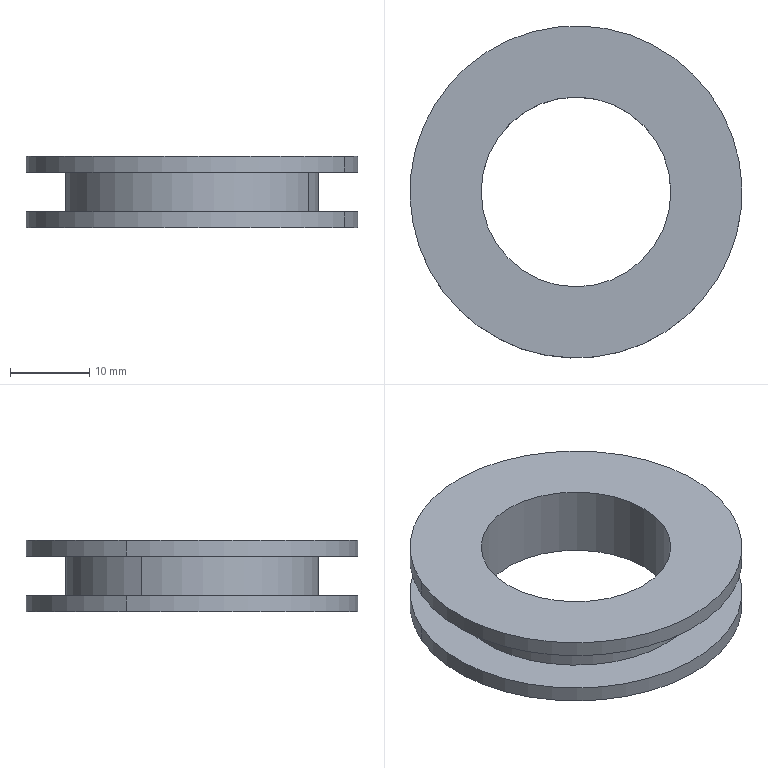Component | SolidWorks | PulleyAssembly-1_Pulley-1 | 1 solid | 12 faces | box 42 x 42 x 9 mm | volume 5492 mm3 | cylinder 8 | plane 4 | commonest cylinder face diameters 42 x4 32 x2 24 x2
build123d program:
from build123d import *


with BuildPart() as part:
    # Sketch1 → Revolve1 (revolve)
    with BuildSketch(Plane(origin=(0, 0, 0), x_dir=(1, 0, 0), z_dir=(0, 1, 0)), mode=Mode.PRIVATE) as revolve1_sk:
        Polygon((12, 4.5), (21, 4.5), (21, 2.5), (16, 2.5), (16, -2.5), (21, -2.5), (21, -4.5), (12, -4.5), align=None)
    revolve(revolve1_sk.sketch.rotate(Axis((0, 0, -4.95), (0, 0, 1)), 180), axis=Axis((0, 0, -4.95), (0, 0, 1)))


solid = part.part

# Placed as in the assembly
solid = solid.moved(Location((-354.55, -345.434, 489.481), (0, 0, 0)))
STEP:
#1=CARTESIAN_POINT('',(-14.718,-13.273,19.094));
#2=VERTEX_POINT('',#1);
#3=CARTESIAN_POINT('',(-13.199,-13.927,19.094));
#4=VERTEX_POINT('',#3);
#5=CARTESIAN_POINT('',(-13.959,-13.6,19.094));
#6=DIRECTION('',(-0.,0.,1.));
#7=DIRECTION('',(-0.9185,0.3954,0.));
#8=AXIS2_PLACEMENT_3D('',#5,#6,#7);
#9=CIRCLE('',#8,0.8268);
#10=EDGE_CURVE('',#2,#4,#9,.T.);
#11=ORIENTED_EDGE('',*,*,#10,.T.);
#12=CARTESIAN_POINT('',(-13.199,-13.927,19.172));
#13=VERTEX_POINT('',#12);
#14=CARTESIAN_POINT('',(-13.199,-13.927,19.466));
#15=DIRECTION('',(-0.,0.,1.));
#16=VECTOR('',#15,39.37);
#17=LINE('',#14,#16);
#18=EDGE_CURVE('',#4,#13,#17,.T.);
#19=ORIENTED_EDGE('',*,*,#18,.T.);
#20=CARTESIAN_POINT('',(-14.718,-13.273,19.172));
#21=VERTEX_POINT('',#20);
#22=CARTESIAN_POINT('',(-13.959,-13.6,19.172));
#23=DIRECTION('',(-0.,0.,1.));
#24=DIRECTION('',(-0.9185,0.3954,0.));
#25=AXIS2_PLACEMENT_3D('',#22,#23,#24);
#26=CIRCLE('',#25,0.8268);
#27=EDGE_CURVE('',#21,#13,#26,.T.);
#28=ORIENTED_EDGE('',*,*,#27,.F.);
#29=CARTESIAN_POINT('',(-14.718,-13.273,19.466));
#30=DIRECTION('',(-0.,0.,1.));
#31=VECTOR('',#30,39.37);
#32=LINE('',#29,#31);
#33=EDGE_CURVE('',#2,#21,#32,.T.);
#34=ORIENTED_EDGE('',*,*,#33,.F.);
#35=EDGE_LOOP('',(#11,#19,#28,#34));
#36=FACE_OUTER_BOUND('',#35,.T.);
#37=CARTESIAN_POINT('',(-13.959,-13.6,19.466));
#38=DIRECTION('',(-0.,0.,1.));
#39=DIRECTION('',(-0.9185,0.3954,0.));
#40=AXIS2_PLACEMENT_3D('',#37,#38,#39);
#41=CYLINDRICAL_SURFACE('',#40,0.8268);
#42=ADVANCED_FACE('',(#36),#41,.T.);
#43=CARTESIAN_POINT('',(-14.537,-13.351,19.172));
#44=VERTEX_POINT('',#43);
#45=CARTESIAN_POINT('',(-13.38,-13.849,19.172));
#46=VERTEX_POINT('',#45);
#47=CARTESIAN_POINT('',(-13.959,-13.6,19.172));
#48=DIRECTION('',(-0.,0.,1.));
#49=DIRECTION('',(-0.9185,0.3954,0.));
#50=AXIS2_PLACEMENT_3D('',#47,#48,#49);
#51=CIRCLE('',#50,0.6299);
#52=EDGE_CURVE('',#44,#46,#51,.T.);
#53=ORIENTED_EDGE('',*,*,#52,.T.);
#54=CARTESIAN_POINT('',(-13.38,-13.849,19.369));
#55=VERTEX_POINT('',#54);
#56=CARTESIAN_POINT('',(-13.38,-13.849,19.466));
#57=DIRECTION('',(-0.,0.,1.));
#58=VECTOR('',#57,39.37);
#59=LINE('',#56,#58);
#60=EDGE_CURVE('',#46,#55,#59,.T.);
#61=ORIENTED_EDGE('',*,*,#60,.T.);
#62=CARTESIAN_POINT('',(-14.537,-13.351,19.369));
#63=VERTEX_POINT('',#62);
#64=CARTESIAN_POINT('',(-13.959,-13.6,19.369));
#65=DIRECTION('',(-0.,0.,1.));
#66=DIRECTION('',(-0.9185,0.3954,0.));
#67=AXIS2_PLACEMENT_3D('',#64,#65,#66);
#68=CIRCLE('',#67,0.6299);
#69=EDGE_CURVE('',#63,#55,#68,.T.);
#70=ORIENTED_EDGE('',*,*,#69,.F.);
#71=CARTESIAN_POINT('',(-14.537,-13.351,19.466));
#72=DIRECTION('',(-0.,0.,1.));
#73=VECTOR('',#72,39.37);
#74=LINE('',#71,#73);
#75=EDGE_CURVE('',#44,#63,#74,.T.);
#76=ORIENTED_EDGE('',*,*,#75,.F.);
#77=EDGE_LOOP('',(#53,#61,#70,#76));
#78=FACE_OUTER_BOUND('',#77,.T.);
#79=CARTESIAN_POINT('',(-13.959,-13.6,19.466));
#80=DIRECTION('',(-0.,0.,1.));
#81=DIRECTION('',(-0.9185,0.3954,0.));
#82=AXIS2_PLACEMENT_3D('',#79,#80,#81);
#83=CYLINDRICAL_SURFACE('',#82,0.6299);
#84=ADVANCED_FACE('',(#78),#83,.T.);
#85=CARTESIAN_POINT('',(-14.718,-13.273,19.369));
#86=VERTEX_POINT('',#85);
#87=CARTESIAN_POINT('',(-13.199,-13.927,19.369));
#88=VERTEX_POINT('',#87);
#89=CARTESIAN_POINT('',(-13.959,-13.6,19.369));
#90=DIRECTION('',(-0.,0.,1.));
#91=DIRECTION('',(-0.9185,0.3954,0.));
#92=AXIS2_PLACEMENT_3D('',#89,#90,#91);
#93=CIRCLE('',#92,0.8268);
#94=EDGE_CURVE('',#86,#88,#93,.T.);
#95=ORIENTED_EDGE('',*,*,#94,.T.);
#96=CARTESIAN_POINT('',(-13.199,-13.927,19.448));
#97=VERTEX_POINT('',#96);
#98=CARTESIAN_POINT('',(-13.199,-13.927,19.466));
#99=DIRECTION('',(-0.,0.,1.));
#100=VECTOR('',#99,39.37);
#101=LINE('',#98,#100);
#102=EDGE_CURVE('',#88,#97,#101,.T.);
#103=ORIENTED_EDGE('',*,*,#102,.T.);
#104=CARTESIAN_POINT('',(-14.718,-13.273,19.448));
#105=VERTEX_POINT('',#104);
#106=CARTESIAN_POINT('',(-13.959,-13.6,19.448));
#107=DIRECTION('',(-0.,0.,1.));
#108=DIRECTION('',(-0.9185,0.3954,0.));
#109=AXIS2_PLACEMENT_3D('',#106,#107,#108);
#110=CIRCLE('',#109,0.8268);
#111=EDGE_CURVE('',#105,#97,#110,.T.);
#112=ORIENTED_EDGE('',*,*,#111,.F.);
#113=CARTESIAN_POINT('',(-14.718,-13.273,19.466));
#114=DIRECTION('',(-0.,0.,1.));
#115=VECTOR('',#114,39.37);
#116=LINE('',#113,#115);
#117=EDGE_CURVE('',#86,#105,#116,.T.);
#118=ORIENTED_EDGE('',*,*,#117,.F.);
#119=EDGE_LOOP('',(#95,#103,#112,#118));
#120=FACE_OUTER_BOUND('',#119,.T.);
#121=CARTESIAN_POINT('',(-13.959,-13.6,19.466));
#122=DIRECTION('',(-0.,0.,1.));
#123=DIRECTION('',(-0.9185,0.3954,0.));
#124=AXIS2_PLACEMENT_3D('',#121,#122,#123);
#125=CYLINDRICAL_SURFACE('',#124,0.8268);
#126=ADVANCED_FACE('',(#120),#125,.T.);
#127=CARTESIAN_POINT('',(-13.525,-13.787,19.094));
#128=VERTEX_POINT('',#127);
#129=CARTESIAN_POINT('',(-14.393,-13.413,19.094));
#130=VERTEX_POINT('',#129);
#131=CARTESIAN_POINT('',(-13.959,-13.6,19.094));
#132=DIRECTION('',(-0.,0.,1.));
#133=DIRECTION('',(-0.9185,0.3954,0.));
#134=AXIS2_PLACEMENT_3D('',#131,#132,#133);
#135=CIRCLE('',#134,0.4724);
#136=EDGE_CURVE('',#128,#130,#135,.T.);
#137=ORIENTED_EDGE('',*,*,#136,.F.);
#138=CARTESIAN_POINT('',(-13.525,-13.787,19.448));
#139=VERTEX_POINT('',#138);
#140=CARTESIAN_POINT('',(-13.525,-13.787,19.466));
#141=DIRECTION('',(-0.,0.,1.));
#142=VECTOR('',#141,39.37);
#143=LINE('',#140,#142);
#144=EDGE_CURVE('',#128,#139,#143,.T.);
#145=ORIENTED_EDGE('',*,*,#144,.T.);
#146=CARTESIAN_POINT('',(-14.393,-13.413,19.448));
#147=VERTEX_POINT('',#146);
#148=CARTESIAN_POINT('',(-13.959,-13.6,19.448));
#149=DIRECTION('',(-0.,0.,1.));
#150=DIRECTION('',(-0.9185,0.3954,0.));
#151=AXIS2_PLACEMENT_3D('',#148,#149,#150);
#152=CIRCLE('',#151,0.4724);
#153=EDGE_CURVE('',#139,#147,#152,.T.);
#154=ORIENTED_EDGE('',*,*,#153,.T.);
#155=CARTESIAN_POINT('',(-14.393,-13.413,19.466));
#156=DIRECTION('',(-0.,0.,1.));
#157=VECTOR('',#156,39.37);
#158=LINE('',#155,#157);
#159=EDGE_CURVE('',#130,#147,#158,.T.);
#160=ORIENTED_EDGE('',*,*,#159,.F.);
#161=EDGE_LOOP('',(#137,#145,#154,#160));
#162=FACE_OUTER_BOUND('',#161,.T.);
#163=CARTESIAN_POINT('',(-13.959,-13.6,19.466));
#164=DIRECTION('',(-0.,0.,1.));
#165=DIRECTION('',(-0.9185,0.3954,0.));
#166=AXIS2_PLACEMENT_3D('',#163,#164,#165);
#167=CYLINDRICAL_SURFACE('',#166,0.4724);
#168=ADVANCED_FACE('',(#162),#167,.F.);
#169=ORIENTED_EDGE('',*,*,#144,.F.);
#170=CARTESIAN_POINT('',(-13.959,-13.6,19.094));
#171=DIRECTION('',(-0.,0.,1.));
#172=DIRECTION('',(-0.9185,0.3954,0.));
#173=AXIS2_PLACEMENT_3D('',#170,#171,#172);
#174=CIRCLE('',#173,0.4724);
#175=EDGE_CURVE('',#130,#128,#174,.T.);
#176=ORIENTED_EDGE('',*,*,#175,.F.);
#177=ORIENTED_EDGE('',*,*,#159,.T.);
#178=CARTESIAN_POINT('',(-13.959,-13.6,19.448));
#179=DIRECTION('',(-0.,0.,1.));
#180=DIRECTION('',(-0.9185,0.3954,0.));
#181=AXIS2_PLACEMENT_3D('',#178,#179,#180);
#182=CIRCLE('',#181,0.4724);
#183=EDGE_CURVE('',#147,#139,#182,.T.);
#184=ORIENTED_EDGE('',*,*,#183,.T.);
#185=EDGE_LOOP('',(#169,#176,#177,#184));
#186=FACE_OUTER_BOUND('',#185,.T.);
#187=CARTESIAN_POINT('',(-13.959,-13.6,19.466));
#188=DIRECTION('',(-0.,0.,1.));
#189=DIRECTION('',(-0.9185,0.3954,0.));
#190=AXIS2_PLACEMENT_3D('',#187,#188,#189);
#191=CYLINDRICAL_SURFACE('',#190,0.4724);
#192=ADVANCED_FACE('',(#186),#191,.F.);
#193=ORIENTED_EDGE('',*,*,#183,.F.);
#194=ORIENTED_EDGE('',*,*,#153,.F.);
#195=EDGE_LOOP('',(#193,#194));
#196=FACE_BOUND('',#195,.T.);
#197=ORIENTED_EDGE('',*,*,#111,.T.);
#198=CARTESIAN_POINT('',(-13.959,-13.6,19.448));
#199=DIRECTION('',(-0.,0.,1.));
#200=DIRECTION('',(-0.9185,0.3954,0.));
#201=AXIS2_PLACEMENT_3D('',#198,#199,#200);
#202=CIRCLE('',#201,0.8268);
#203=EDGE_CURVE('',#97,#105,#202,.T.);
#204=ORIENTED_EDGE('',*,*,#203,.T.);
#205=EDGE_LOOP('',(#197,#204));
#206=FACE_OUTER_BOUND('',#205,.T.);
#207=CARTESIAN_POINT('',(-13.525,-13.787,19.448));
#208=DIRECTION('',(0.,-0.,-1.));
#209=DIRECTION('',(0.9185,-0.3954,0.));
#210=AXIS2_PLACEMENT_3D('',#207,#208,#209);
#211=PLANE('',#210);
#212=ADVANCED_FACE('',(#196,#206),#211,.F.);
#213=ORIENTED_EDGE('',*,*,#102,.F.);
#214=CARTESIAN_POINT('',(-13.959,-13.6,19.369));
#215=DIRECTION('',(-0.,0.,1.));
#216=DIRECTION('',(-0.9185,0.3954,0.));
#217=AXIS2_PLACEMENT_3D('',#214,#215,#216);
#218=CIRCLE('',#217,0.8268);
#219=EDGE_CURVE('',#88,#86,#218,.T.);
#220=ORIENTED_EDGE('',*,*,#219,.T.);
#221=ORIENTED_EDGE('',*,*,#117,.T.);
#222=ORIENTED_EDGE('',*,*,#203,.F.);
#223=EDGE_LOOP('',(#213,#220,#221,#222));
#224=FACE_OUTER_BOUND('',#223,.T.);
#225=CARTESIAN_POINT('',(-13.959,-13.6,19.466));
#226=DIRECTION('',(-0.,0.,1.));
#227=DIRECTION('',(-0.9185,0.3954,0.));
#228=AXIS2_PLACEMENT_3D('',#225,#226,#227);
#229=CYLINDRICAL_SURFACE('',#228,0.8268);
#230=ADVANCED_FACE('',(#224),#229,.T.);
#231=ORIENTED_EDGE('',*,*,#94,.F.);
#232=ORIENTED_EDGE('',*,*,#219,.F.);
#233=EDGE_LOOP('',(#231,#232));
#234=FACE_OUTER_BOUND('',#233,.T.);
#235=ORIENTED_EDGE('',*,*,#69,.T.);
#236=CARTESIAN_POINT('',(-13.959,-13.6,19.369));
#237=DIRECTION('',(-0.,0.,1.));
#238=DIRECTION('',(-0.9185,0.3954,0.));
#239=AXIS2_PLACEMENT_3D('',#236,#237,#238);
#240=CIRCLE('',#239,0.6299);
#241=EDGE_CURVE('',#55,#63,#240,.T.);
#242=ORIENTED_EDGE('',*,*,#241,.T.);
#243=EDGE_LOOP('',(#235,#242));
#244=FACE_BOUND('',#243,.T.);
#245=CARTESIAN_POINT('',(-13.199,-13.927,19.369));
#246=DIRECTION('',(-0.,0.,1.));
#247=DIRECTION('',(-0.9185,0.3954,-0.));
#248=AXIS2_PLACEMENT_3D('',#245,#246,#247);
#249=PLANE('',#248);
#250=ADVANCED_FACE('',(#234,#244),#249,.F.);
#251=ORIENTED_EDGE('',*,*,#60,.F.);
#252=CARTESIAN_POINT('',(-13.959,-13.6,19.172));
#253=DIRECTION('',(-0.,0.,1.));
#254=DIRECTION('',(-0.9185,0.3954,0.));
#255=AXIS2_PLACEMENT_3D('',#252,#253,#254);
#256=CIRCLE('',#255,0.6299);
#257=EDGE_CURVE('',#46,#44,#256,.T.);
#258=ORIENTED_EDGE('',*,*,#257,.T.);
#259=ORIENTED_EDGE('',*,*,#75,.T.);
#260=ORIENTED_EDGE('',*,*,#241,.F.);
#261=EDGE_LOOP('',(#251,#258,#259,#260));
#262=FACE_OUTER_BOUND('',#261,.T.);
#263=CARTESIAN_POINT('',(-13.959,-13.6,19.466));
#264=DIRECTION('',(-0.,0.,1.));
#265=DIRECTION('',(-0.9185,0.3954,0.));
#266=AXIS2_PLACEMENT_3D('',#263,#264,#265);
#267=CYLINDRICAL_SURFACE('',#266,0.6299);
#268=ADVANCED_FACE('',(#262),#267,.T.);
#269=ORIENTED_EDGE('',*,*,#52,.F.);
#270=ORIENTED_EDGE('',*,*,#257,.F.);
#271=EDGE_LOOP('',(#269,#270));
#272=FACE_BOUND('',#271,.T.);
#273=ORIENTED_EDGE('',*,*,#27,.T.);
#274=CARTESIAN_POINT('',(-13.959,-13.6,19.172));
#275=DIRECTION('',(-0.,0.,1.));
#276=DIRECTION('',(-0.9185,0.3954,0.));
#277=AXIS2_PLACEMENT_3D('',#274,#275,#276);
#278=CIRCLE('',#277,0.8268);
#279=EDGE_CURVE('',#13,#21,#278,.T.);
#280=ORIENTED_EDGE('',*,*,#279,.T.);
#281=EDGE_LOOP('',(#273,#280));
#282=FACE_OUTER_BOUND('',#281,.T.);
#283=CARTESIAN_POINT('',(-13.38,-13.849,19.172));
#284=DIRECTION('',(0.,-0.,-1.));
#285=DIRECTION('',(0.9185,-0.3954,0.));
#286=AXIS2_PLACEMENT_3D('',#283,#284,#285);
#287=PLANE('',#286);
#288=ADVANCED_FACE('',(#272,#282),#287,.F.);
#289=ORIENTED_EDGE('',*,*,#18,.F.);
#290=CARTESIAN_POINT('',(-13.959,-13.6,19.094));
#291=DIRECTION('',(-0.,0.,1.));
#292=DIRECTION('',(-0.9185,0.3954,0.));
#293=AXIS2_PLACEMENT_3D('',#290,#291,#292);
#294=CIRCLE('',#293,0.8268);
#295=EDGE_CURVE('',#4,#2,#294,.T.);
#296=ORIENTED_EDGE('',*,*,#295,.T.);
#297=ORIENTED_EDGE('',*,*,#33,.T.);
#298=ORIENTED_EDGE('',*,*,#279,.F.);
#299=EDGE_LOOP('',(#289,#296,#297,#298));
#300=FACE_OUTER_BOUND('',#299,.T.);
#301=CARTESIAN_POINT('',(-13.959,-13.6,19.466));
#302=DIRECTION('',(-0.,0.,1.));
#303=DIRECTION('',(-0.9185,0.3954,0.));
#304=AXIS2_PLACEMENT_3D('',#301,#302,#303);
#305=CYLINDRICAL_SURFACE('',#304,0.8268);
#306=ADVANCED_FACE('',(#300),#305,.T.);
#307=ORIENTED_EDGE('',*,*,#10,.F.);
#308=ORIENTED_EDGE('',*,*,#295,.F.);
#309=EDGE_LOOP('',(#307,#308));
#310=FACE_OUTER_BOUND('',#309,.T.);
#311=ORIENTED_EDGE('',*,*,#175,.T.);
#312=ORIENTED_EDGE('',*,*,#136,.T.);
#313=EDGE_LOOP('',(#311,#312));
#314=FACE_BOUND('',#313,.T.);
#315=CARTESIAN_POINT('',(-13.199,-13.927,19.094));
#316=DIRECTION('',(-0.,0.,1.));
#317=DIRECTION('',(-0.9185,0.3954,-0.));
#318=AXIS2_PLACEMENT_3D('',#315,#316,#317);
#319=PLANE('',#318);
#320=ADVANCED_FACE('',(#310,#314),#319,.F.);
#321=CLOSED_SHELL('',(#42,#84,#126,#168,#192,#212,#230,#250,#268,#288,#306,#320));
#322=MANIFOLD_SOLID_BREP('',#321);
#323=CARTESIAN_POINT('',(0.,0.,0.));
#324=DIRECTION('',(0.,0.,1.));
#325=DIRECTION('',(1.,0.,0.));
#326=AXIS2_PLACEMENT_3D('',#323,#324,#325);
#327=(LENGTH_UNIT()NAMED_UNIT(*)SI_UNIT($,.METRE.));
#328=LENGTH_MEASURE_WITH_UNIT(LENGTH_MEASURE(0.0254),#327);
#329=DIMENSIONAL_EXPONENTS(1.,0.,0.,0.,0.,0.,0.);
#330=(CONVERSION_BASED_UNIT('',#328)LENGTH_UNIT()NAMED_UNIT(#329));
#331=UNCERTAINTY_MEASURE_WITH_UNIT(LENGTH_MEASURE(0.00001),#330,'','');
#332=(NAMED_UNIT(*)PLANE_ANGLE_UNIT()SI_UNIT($,.RADIAN.));
#333=(NAMED_UNIT(*)SI_UNIT($,.STERADIAN.)SOLID_ANGLE_UNIT());
#334=(GEOMETRIC_REPRESENTATION_CONTEXT(3)GLOBAL_UNCERTAINTY_ASSIGNED_CONTEXT((#331))GLOBAL_UNIT_ASSIGNED_CONTEXT((#330,#332,#333))REPRESENTATION_CONTEXT('',''));
#335=ADVANCED_BREP_SHAPE_REPRESENTATION('',(#322,#326),#334);
#336=COLOUR_RGB('',0.7922,0.8196,0.9333);
#337=FILL_AREA_STYLE_COLOUR('',#336);
#338=FILL_AREA_STYLE('',(#337));
#339=SURFACE_STYLE_FILL_AREA(#338);
#340=SURFACE_SIDE_STYLE('',(#339));
#341=SURFACE_STYLE_USAGE(.BOTH.,#340);
#342=PRESENTATION_STYLE_ASSIGNMENT((#341));
#343=STYLED_ITEM('',(#342),#322);
#344=(LENGTH_UNIT()NAMED_UNIT(*)SI_UNIT($,.METRE.));
#345=LENGTH_MEASURE_WITH_UNIT(LENGTH_MEASURE(0.0254),#344);
#346=DIMENSIONAL_EXPONENTS(1.,0.,0.,0.,0.,0.,0.);
#347=(CONVERSION_BASED_UNIT('',#345)LENGTH_UNIT()NAMED_UNIT(#346));
#348=UNCERTAINTY_MEASURE_WITH_UNIT(LENGTH_MEASURE(0.00001),#347,'','');
#349=(NAMED_UNIT(*)PLANE_ANGLE_UNIT()SI_UNIT($,.RADIAN.));
#350=(NAMED_UNIT(*)SI_UNIT($,.STERADIAN.)SOLID_ANGLE_UNIT());
#351=(GEOMETRIC_REPRESENTATION_CONTEXT(3)GLOBAL_UNCERTAINTY_ASSIGNED_CONTEXT((#348))GLOBAL_UNIT_ASSIGNED_CONTEXT((#347,#349,#350))REPRESENTATION_CONTEXT('',''));
#352=MECHANICAL_DESIGN_GEOMETRIC_PRESENTATION_REPRESENTATION('',(#343),#351);
#353=PRESENTATION_LAYER_ASSIGNMENT('','',(#343));